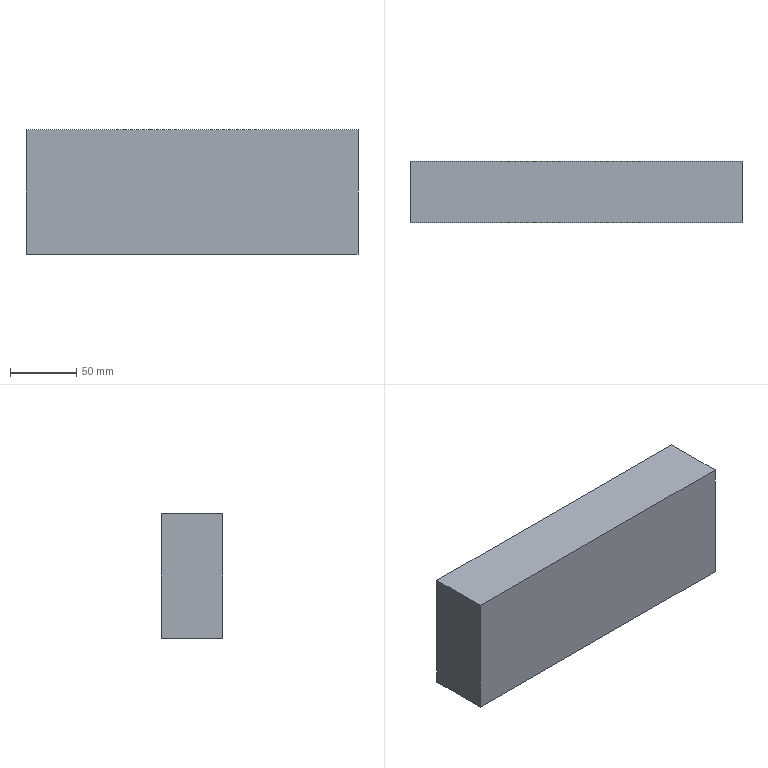Component | SolidWorks | FixedFrame-1 | 1 solid | 22 faces | box 250 x 46.3 x 93.8 mm | volume 1084835 mm3 | plane 14 | cylinder 8 | commonest cylinder face diameters 5 x8
build123d program:
from build123d import *

# Parameters (mm, degrees)
SKETCH2_2_W         = 250
SKETCH2_2_H         = 93.801
BOSS_EXTRUDE1_DEPTH = 44
MOVE_FACE1_BY       = 2.3
SKETCH1_R           = 2.5
CUT_EXTRUDE1_DEPTH  = 8
SKETCH2_W           = 22
SKETCH2_H           = 11
CUT_EXTRUDE2_DEPTH  = 1.5


with BuildPart() as part:
    # Sketch2_2 → Boss-Extrude1 (new body)
    with BuildSketch(Plane.XY):
        with Locations((0, 780.702)):
            Rectangle(SKETCH2_2_W, SKETCH2_2_H)
    extrude(amount=BOSS_EXTRUDE1_DEPTH)

    # Move Face1: a face moved outward by 2.3
    extrude(part.faces().sort_by_distance((0, 780.702, 44))[0], amount=MOVE_FACE1_BY, dir=(0, 0, 1))

    # Sketch1 → Cut-Extrude1 (cut)
    with BuildSketch(Plane.XY.offset(46.3)):
        with Locations((31.25, 802.301)):
            Circle(SKETCH1_R)
        with Locations((31.25, 752.301)):
            Circle(SKETCH1_R)
        with Locations((-31.25, 752.301)):
            Circle(SKETCH1_R)
        with Locations((-31.25, 802.301)):
            Circle(SKETCH1_R)
    extrude(amount=-CUT_EXTRUDE1_DEPTH, mode=Mode.SUBTRACT)

    # Sketch2 → Cut-Extrude2 (cut)
    with BuildSketch(Plane.XY.offset(46.3)):
        with Locations((0, 824.5)):
            Rectangle(SKETCH2_W, SKETCH2_H)
    extrude(amount=-CUT_EXTRUDE2_DEPTH, mode=Mode.SUBTRACT)


solid = part.part

# Placed as in the assembly
solid = solid.moved(Location((0, -295.035, 48), (-90, 0, 0)))
STEP:
#1=CARTESIAN_POINT('',(-1.329,-10.108,-29.697));
#2=VERTEX_POINT('',#1);
#3=CARTESIAN_POINT('',(-1.132,-10.108,-29.697));
#4=VERTEX_POINT('',#3);
#5=CARTESIAN_POINT('',(-1.23,-10.108,-29.697));
#6=DIRECTION('',(0.,1.,0.));
#7=DIRECTION('',(1.,0.,0.));
#8=AXIS2_PLACEMENT_3D('',#5,#6,#7);
#9=CIRCLE('',#8,0.09843);
#10=EDGE_CURVE('',#2,#4,#9,.T.);
#11=ORIENTED_EDGE('',*,*,#10,.F.);
#12=CARTESIAN_POINT('',(-1.329,-9.793,-29.697));
#13=VERTEX_POINT('',#12);
#14=CARTESIAN_POINT('',(-1.329,-10.108,-29.697));
#15=DIRECTION('',(0.,1.,0.));
#16=VECTOR('',#15,39.37);
#17=LINE('',#14,#16);
#18=EDGE_CURVE('',#2,#13,#17,.T.);
#19=ORIENTED_EDGE('',*,*,#18,.T.);
#20=CARTESIAN_POINT('',(-1.132,-9.793,-29.697));
#21=VERTEX_POINT('',#20);
#22=CARTESIAN_POINT('',(-1.23,-9.793,-29.697));
#23=DIRECTION('',(0.,1.,0.));
#24=DIRECTION('',(1.,0.,0.));
#25=AXIS2_PLACEMENT_3D('',#22,#23,#24);
#26=CIRCLE('',#25,0.09843);
#27=EDGE_CURVE('',#13,#21,#26,.T.);
#28=ORIENTED_EDGE('',*,*,#27,.T.);
#29=CARTESIAN_POINT('',(-1.132,-10.108,-29.697));
#30=DIRECTION('',(0.,1.,0.));
#31=VECTOR('',#30,39.37);
#32=LINE('',#29,#31);
#33=EDGE_CURVE('',#4,#21,#32,.T.);
#34=ORIENTED_EDGE('',*,*,#33,.F.);
#35=EDGE_LOOP('',(#11,#19,#28,#34));
#36=FACE_OUTER_BOUND('',#35,.T.);
#37=CARTESIAN_POINT('',(-1.23,-10.108,-29.697));
#38=DIRECTION('',(0.,1.,0.));
#39=DIRECTION('',(1.,0.,0.));
#40=AXIS2_PLACEMENT_3D('',#37,#38,#39);
#41=CYLINDRICAL_SURFACE('',#40,0.09843);
#42=ADVANCED_FACE('',(#36),#41,.F.);
#43=CARTESIAN_POINT('',(-1.329,-10.108,-27.728));
#44=VERTEX_POINT('',#43);
#45=CARTESIAN_POINT('',(-1.132,-10.108,-27.728));
#46=VERTEX_POINT('',#45);
#47=CARTESIAN_POINT('',(-1.23,-10.108,-27.728));
#48=DIRECTION('',(0.,1.,0.));
#49=DIRECTION('',(1.,0.,0.));
#50=AXIS2_PLACEMENT_3D('',#47,#48,#49);
#51=CIRCLE('',#50,0.09843);
#52=EDGE_CURVE('',#44,#46,#51,.T.);
#53=ORIENTED_EDGE('',*,*,#52,.F.);
#54=CARTESIAN_POINT('',(-1.329,-9.793,-27.728));
#55=VERTEX_POINT('',#54);
#56=CARTESIAN_POINT('',(-1.329,-10.108,-27.728));
#57=DIRECTION('',(0.,1.,0.));
#58=VECTOR('',#57,39.37);
#59=LINE('',#56,#58);
#60=EDGE_CURVE('',#44,#55,#59,.T.);
#61=ORIENTED_EDGE('',*,*,#60,.T.);
#62=CARTESIAN_POINT('',(-1.132,-9.793,-27.728));
#63=VERTEX_POINT('',#62);
#64=CARTESIAN_POINT('',(-1.23,-9.793,-27.728));
#65=DIRECTION('',(0.,1.,0.));
#66=DIRECTION('',(1.,0.,0.));
#67=AXIS2_PLACEMENT_3D('',#64,#65,#66);
#68=CIRCLE('',#67,0.09843);
#69=EDGE_CURVE('',#55,#63,#68,.T.);
#70=ORIENTED_EDGE('',*,*,#69,.T.);
#71=CARTESIAN_POINT('',(-1.132,-10.108,-27.728));
#72=DIRECTION('',(0.,1.,0.));
#73=VECTOR('',#72,39.37);
#74=LINE('',#71,#73);
#75=EDGE_CURVE('',#46,#63,#74,.T.);
#76=ORIENTED_EDGE('',*,*,#75,.F.);
#77=EDGE_LOOP('',(#53,#61,#70,#76));
#78=FACE_OUTER_BOUND('',#77,.T.);
#79=CARTESIAN_POINT('',(-1.23,-10.108,-27.728));
#80=DIRECTION('',(0.,1.,0.));
#81=DIRECTION('',(1.,0.,0.));
#82=AXIS2_PLACEMENT_3D('',#79,#80,#81);
#83=CYLINDRICAL_SURFACE('',#82,0.09843);
#84=ADVANCED_FACE('',(#78),#83,.F.);
#85=CARTESIAN_POINT('',(1.132,-10.108,-27.728));
#86=VERTEX_POINT('',#85);
#87=CARTESIAN_POINT('',(1.329,-10.108,-27.728));
#88=VERTEX_POINT('',#87);
#89=CARTESIAN_POINT('',(1.23,-10.108,-27.728));
#90=DIRECTION('',(0.,1.,0.));
#91=DIRECTION('',(1.,0.,0.));
#92=AXIS2_PLACEMENT_3D('',#89,#90,#91);
#93=CIRCLE('',#92,0.09843);
#94=EDGE_CURVE('',#86,#88,#93,.T.);
#95=ORIENTED_EDGE('',*,*,#94,.F.);
#96=CARTESIAN_POINT('',(1.132,-9.793,-27.728));
#97=VERTEX_POINT('',#96);
#98=CARTESIAN_POINT('',(1.132,-10.108,-27.728));
#99=DIRECTION('',(0.,1.,0.));
#100=VECTOR('',#99,39.37);
#101=LINE('',#98,#100);
#102=EDGE_CURVE('',#86,#97,#101,.T.);
#103=ORIENTED_EDGE('',*,*,#102,.T.);
#104=CARTESIAN_POINT('',(1.329,-9.793,-27.728));
#105=VERTEX_POINT('',#104);
#106=CARTESIAN_POINT('',(1.23,-9.793,-27.728));
#107=DIRECTION('',(0.,1.,0.));
#108=DIRECTION('',(1.,0.,0.));
#109=AXIS2_PLACEMENT_3D('',#106,#107,#108);
#110=CIRCLE('',#109,0.09843);
#111=EDGE_CURVE('',#97,#105,#110,.T.);
#112=ORIENTED_EDGE('',*,*,#111,.T.);
#113=CARTESIAN_POINT('',(1.329,-10.108,-27.728));
#114=DIRECTION('',(0.,1.,0.));
#115=VECTOR('',#114,39.37);
#116=LINE('',#113,#115);
#117=EDGE_CURVE('',#88,#105,#116,.T.);
#118=ORIENTED_EDGE('',*,*,#117,.F.);
#119=EDGE_LOOP('',(#95,#103,#112,#118));
#120=FACE_OUTER_BOUND('',#119,.T.);
#121=CARTESIAN_POINT('',(1.23,-10.108,-27.728));
#122=DIRECTION('',(0.,1.,0.));
#123=DIRECTION('',(1.,0.,0.));
#124=AXIS2_PLACEMENT_3D('',#121,#122,#123);
#125=CYLINDRICAL_SURFACE('',#124,0.09843);
#126=ADVANCED_FACE('',(#120),#125,.F.);
#127=CARTESIAN_POINT('',(1.132,-10.108,-29.697));
#128=VERTEX_POINT('',#127);
#129=CARTESIAN_POINT('',(1.329,-10.108,-29.697));
#130=VERTEX_POINT('',#129);
#131=CARTESIAN_POINT('',(1.23,-10.108,-29.697));
#132=DIRECTION('',(0.,1.,0.));
#133=DIRECTION('',(1.,0.,0.));
#134=AXIS2_PLACEMENT_3D('',#131,#132,#133);
#135=CIRCLE('',#134,0.09843);
#136=EDGE_CURVE('',#128,#130,#135,.T.);
#137=ORIENTED_EDGE('',*,*,#136,.F.);
#138=CARTESIAN_POINT('',(1.132,-9.793,-29.697));
#139=VERTEX_POINT('',#138);
#140=CARTESIAN_POINT('',(1.132,-10.108,-29.697));
#141=DIRECTION('',(0.,1.,0.));
#142=VECTOR('',#141,39.37);
#143=LINE('',#140,#142);
#144=EDGE_CURVE('',#128,#139,#143,.T.);
#145=ORIENTED_EDGE('',*,*,#144,.T.);
#146=CARTESIAN_POINT('',(1.329,-9.793,-29.697));
#147=VERTEX_POINT('',#146);
#148=CARTESIAN_POINT('',(1.23,-9.793,-29.697));
#149=DIRECTION('',(0.,1.,0.));
#150=DIRECTION('',(1.,0.,0.));
#151=AXIS2_PLACEMENT_3D('',#148,#149,#150);
#152=CIRCLE('',#151,0.09843);
#153=EDGE_CURVE('',#139,#147,#152,.T.);
#154=ORIENTED_EDGE('',*,*,#153,.T.);
#155=CARTESIAN_POINT('',(1.329,-10.108,-29.697));
#156=DIRECTION('',(0.,1.,0.));
#157=VECTOR('',#156,39.37);
#158=LINE('',#155,#157);
#159=EDGE_CURVE('',#130,#147,#158,.T.);
#160=ORIENTED_EDGE('',*,*,#159,.F.);
#161=EDGE_LOOP('',(#137,#145,#154,#160));
#162=FACE_OUTER_BOUND('',#161,.T.);
#163=CARTESIAN_POINT('',(1.23,-10.108,-29.697));
#164=DIRECTION('',(0.,1.,0.));
#165=DIRECTION('',(1.,0.,0.));
#166=AXIS2_PLACEMENT_3D('',#163,#164,#165);
#167=CYLINDRICAL_SURFACE('',#166,0.09843);
#168=ADVANCED_FACE('',(#162),#167,.F.);
#169=CARTESIAN_POINT('',(4.921,-11.616,-27.));
#170=VERTEX_POINT('',#169);
#171=CARTESIAN_POINT('',(4.921,-11.616,-30.693));
#172=VERTEX_POINT('',#171);
#173=CARTESIAN_POINT('',(4.921,-11.616,-27.));
#174=DIRECTION('',(0.,0.,-1.));
#175=VECTOR('',#174,39.37);
#176=LINE('',#173,#175);
#177=EDGE_CURVE('',#170,#172,#176,.T.);
#178=ORIENTED_EDGE('',*,*,#177,.T.);
#179=CARTESIAN_POINT('',(4.921,-9.793,-30.693));
#180=VERTEX_POINT('',#179);
#181=CARTESIAN_POINT('',(4.921,-9.883,-30.693));
#182=DIRECTION('',(0.,-1.,0.));
#183=VECTOR('',#182,39.37);
#184=LINE('',#181,#183);
#185=EDGE_CURVE('',#180,#172,#184,.T.);
#186=ORIENTED_EDGE('',*,*,#185,.F.);
#187=CARTESIAN_POINT('',(4.921,-9.793,-27.));
#188=VERTEX_POINT('',#187);
#189=CARTESIAN_POINT('',(4.921,-9.793,-27.));
#190=DIRECTION('',(0.,0.,-1.));
#191=VECTOR('',#190,39.37);
#192=LINE('',#189,#191);
#193=EDGE_CURVE('',#188,#180,#192,.T.);
#194=ORIENTED_EDGE('',*,*,#193,.F.);
#195=CARTESIAN_POINT('',(4.921,-9.883,-27.));
#196=DIRECTION('',(0.,-1.,0.));
#197=VECTOR('',#196,39.37);
#198=LINE('',#195,#197);
#199=EDGE_CURVE('',#188,#170,#198,.T.);
#200=ORIENTED_EDGE('',*,*,#199,.T.);
#201=EDGE_LOOP('',(#178,#186,#194,#200));
#202=FACE_OUTER_BOUND('',#201,.T.);
#203=CARTESIAN_POINT('',(4.921,-9.883,-27.));
#204=DIRECTION('',(-1.,0.,0.));
#205=DIRECTION('',(0.,1.,0.));
#206=AXIS2_PLACEMENT_3D('',#203,#204,#205);
#207=PLANE('',#206);
#208=ADVANCED_FACE('',(#202),#207,.F.);
#209=CARTESIAN_POINT('',(-0.4331,-9.793,-30.693));
#210=VERTEX_POINT('',#209);
#211=CARTESIAN_POINT('',(-4.921,-9.793,-30.693));
#212=VERTEX_POINT('',#211);
#213=CARTESIAN_POINT('',(4.921,-9.793,-30.693));
#214=DIRECTION('',(-1.,0.,0.));
#215=VECTOR('',#214,39.37);
#216=LINE('',#213,#215);
#217=EDGE_CURVE('',#210,#212,#216,.T.);
#218=ORIENTED_EDGE('',*,*,#217,.F.);
#219=CARTESIAN_POINT('',(-0.4331,-9.852,-30.693));
#220=VERTEX_POINT('',#219);
#221=CARTESIAN_POINT('',(-0.4331,-9.883,-30.693));
#222=DIRECTION('',(0.,-1.,0.));
#223=VECTOR('',#222,39.37);
#224=LINE('',#221,#223);
#225=EDGE_CURVE('',#210,#220,#224,.T.);
#226=ORIENTED_EDGE('',*,*,#225,.T.);
#227=CARTESIAN_POINT('',(0.4331,-9.852,-30.693));
#228=VERTEX_POINT('',#227);
#229=CARTESIAN_POINT('',(4.921,-9.852,-30.693));
#230=DIRECTION('',(1.,0.,0.));
#231=VECTOR('',#230,39.37);
#232=LINE('',#229,#231);
#233=EDGE_CURVE('',#220,#228,#232,.T.);
#234=ORIENTED_EDGE('',*,*,#233,.T.);
#235=CARTESIAN_POINT('',(0.4331,-9.793,-30.693));
#236=VERTEX_POINT('',#235);
#237=CARTESIAN_POINT('',(0.4331,-9.883,-30.693));
#238=DIRECTION('',(0.,1.,0.));
#239=VECTOR('',#238,39.37);
#240=LINE('',#237,#239);
#241=EDGE_CURVE('',#228,#236,#240,.T.);
#242=ORIENTED_EDGE('',*,*,#241,.T.);
#243=CARTESIAN_POINT('',(4.921,-9.793,-30.693));
#244=DIRECTION('',(-1.,0.,0.));
#245=VECTOR('',#244,39.37);
#246=LINE('',#243,#245);
#247=EDGE_CURVE('',#180,#236,#246,.T.);
#248=ORIENTED_EDGE('',*,*,#247,.F.);
#249=ORIENTED_EDGE('',*,*,#185,.T.);
#250=CARTESIAN_POINT('',(-4.921,-11.616,-30.693));
#251=VERTEX_POINT('',#250);
#252=CARTESIAN_POINT('',(4.921,-11.616,-30.693));
#253=DIRECTION('',(-1.,0.,0.));
#254=VECTOR('',#253,39.37);
#255=LINE('',#252,#254);
#256=EDGE_CURVE('',#172,#251,#255,.T.);
#257=ORIENTED_EDGE('',*,*,#256,.T.);
#258=CARTESIAN_POINT('',(-4.921,-9.883,-30.693));
#259=DIRECTION('',(0.,-1.,0.));
#260=VECTOR('',#259,39.37);
#261=LINE('',#258,#260);
#262=EDGE_CURVE('',#212,#251,#261,.T.);
#263=ORIENTED_EDGE('',*,*,#262,.F.);
#264=EDGE_LOOP('',(#218,#226,#234,#242,#248,#249,#257,#263));
#265=FACE_OUTER_BOUND('',#264,.T.);
#266=CARTESIAN_POINT('',(4.921,-9.883,-30.693));
#267=DIRECTION('',(0.,0.,1.));
#268=DIRECTION('',(0.,-1.,0.));
#269=AXIS2_PLACEMENT_3D('',#266,#267,#268);
#270=PLANE('',#269);
#271=ADVANCED_FACE('',(#265),#270,.F.);
#272=CARTESIAN_POINT('',(-4.921,-11.616,-27.));
#273=VERTEX_POINT('',#272);
#274=CARTESIAN_POINT('',(-4.921,-11.616,-27.));
#275=DIRECTION('',(0.,0.,1.));
#276=VECTOR('',#275,39.37);
#277=LINE('',#274,#276);
#278=EDGE_CURVE('',#251,#273,#277,.T.);
#279=ORIENTED_EDGE('',*,*,#278,.T.);
#280=CARTESIAN_POINT('',(-4.921,-9.793,-27.));
#281=VERTEX_POINT('',#280);
#282=CARTESIAN_POINT('',(-4.921,-9.883,-27.));
#283=DIRECTION('',(0.,-1.,0.));
#284=VECTOR('',#283,39.37);
#285=LINE('',#282,#284);
#286=EDGE_CURVE('',#281,#273,#285,.T.);
#287=ORIENTED_EDGE('',*,*,#286,.F.);
#288=CARTESIAN_POINT('',(-4.921,-9.793,-27.));
#289=DIRECTION('',(0.,0.,1.));
#290=VECTOR('',#289,39.37);
#291=LINE('',#288,#290);
#292=EDGE_CURVE('',#212,#281,#291,.T.);
#293=ORIENTED_EDGE('',*,*,#292,.F.);
#294=ORIENTED_EDGE('',*,*,#262,.T.);
#295=EDGE_LOOP('',(#279,#287,#293,#294));
#296=FACE_OUTER_BOUND('',#295,.T.);
#297=CARTESIAN_POINT('',(-4.921,-9.883,-27.));
#298=DIRECTION('',(1.,0.,0.));
#299=DIRECTION('',(0.,-1.,0.));
#300=AXIS2_PLACEMENT_3D('',#297,#298,#299);
#301=PLANE('',#300);
#302=ADVANCED_FACE('',(#296),#301,.F.);
#303=CARTESIAN_POINT('',(4.921,-11.616,-27.));
#304=DIRECTION('',(1.,0.,0.));
#305=VECTOR('',#304,39.37);
#306=LINE('',#303,#305);
#307=EDGE_CURVE('',#273,#170,#306,.T.);
#308=ORIENTED_EDGE('',*,*,#307,.T.);
#309=ORIENTED_EDGE('',*,*,#199,.F.);
#310=CARTESIAN_POINT('',(4.921,-9.793,-27.));
#311=DIRECTION('',(1.,0.,0.));
#312=VECTOR('',#311,39.37);
#313=LINE('',#310,#312);
#314=EDGE_CURVE('',#281,#188,#313,.T.);
#315=ORIENTED_EDGE('',*,*,#314,.F.);
#316=ORIENTED_EDGE('',*,*,#286,.T.);
#317=EDGE_LOOP('',(#308,#309,#315,#316));
#318=FACE_OUTER_BOUND('',#317,.T.);
#319=CARTESIAN_POINT('',(4.921,-9.883,-27.));
#320=DIRECTION('',(0.,0.,-1.));
#321=DIRECTION('',(0.,1.,0.));
#322=AXIS2_PLACEMENT_3D('',#319,#320,#321);
#323=PLANE('',#322);
#324=ADVANCED_FACE('',(#318),#323,.F.);
#325=CARTESIAN_POINT('',(-0.4331,-9.793,-30.354));
#326=VERTEX_POINT('',#325);
#327=CARTESIAN_POINT('',(-0.4331,-9.793,-30.354));
#328=DIRECTION('',(0.,0.,1.));
#329=VECTOR('',#328,39.37);
#330=LINE('',#327,#329);
#331=EDGE_CURVE('',#210,#326,#330,.T.);
#332=ORIENTED_EDGE('',*,*,#331,.F.);
#333=ORIENTED_EDGE('',*,*,#217,.T.);
#334=ORIENTED_EDGE('',*,*,#292,.T.);
#335=ORIENTED_EDGE('',*,*,#314,.T.);
#336=ORIENTED_EDGE('',*,*,#193,.T.);
#337=ORIENTED_EDGE('',*,*,#247,.T.);
#338=CARTESIAN_POINT('',(0.4331,-9.793,-30.354));
#339=VERTEX_POINT('',#338);
#340=CARTESIAN_POINT('',(0.4331,-9.793,-30.354));
#341=DIRECTION('',(0.,0.,-1.));
#342=VECTOR('',#341,39.37);
#343=LINE('',#340,#342);
#344=EDGE_CURVE('',#339,#236,#343,.T.);
#345=ORIENTED_EDGE('',*,*,#344,.F.);
#346=CARTESIAN_POINT('',(-0.4331,-9.793,-30.354));
#347=DIRECTION('',(1.,0.,0.));
#348=VECTOR('',#347,39.37);
#349=LINE('',#346,#348);
#350=EDGE_CURVE('',#326,#339,#349,.T.);
#351=ORIENTED_EDGE('',*,*,#350,.F.);
#352=EDGE_LOOP('',(#332,#333,#334,#335,#336,#337,#345,#351));
#353=FACE_OUTER_BOUND('',#352,.T.);
#354=CARTESIAN_POINT('',(-1.23,-9.793,-29.697));
#355=DIRECTION('',(0.,1.,0.));
#356=DIRECTION('',(1.,0.,0.));
#357=AXIS2_PLACEMENT_3D('',#354,#355,#356);
#358=CIRCLE('',#357,0.09843);
#359=EDGE_CURVE('',#21,#13,#358,.T.);
#360=ORIENTED_EDGE('',*,*,#359,.F.);
#361=ORIENTED_EDGE('',*,*,#27,.F.);
#362=EDGE_LOOP('',(#360,#361));
#363=FACE_BOUND('',#362,.T.);
#364=CARTESIAN_POINT('',(-1.23,-9.793,-27.728));
#365=DIRECTION('',(0.,1.,0.));
#366=DIRECTION('',(1.,0.,0.));
#367=AXIS2_PLACEMENT_3D('',#364,#365,#366);
#368=CIRCLE('',#367,0.09843);
#369=EDGE_CURVE('',#63,#55,#368,.T.);
#370=ORIENTED_EDGE('',*,*,#369,.F.);
#371=ORIENTED_EDGE('',*,*,#69,.F.);
#372=EDGE_LOOP('',(#370,#371));
#373=FACE_BOUND('',#372,.T.);
#374=CARTESIAN_POINT('',(1.23,-9.793,-27.728));
#375=DIRECTION('',(0.,1.,0.));
#376=DIRECTION('',(1.,0.,0.));
#377=AXIS2_PLACEMENT_3D('',#374,#375,#376);
#378=CIRCLE('',#377,0.09843);
#379=EDGE_CURVE('',#105,#97,#378,.T.);
#380=ORIENTED_EDGE('',*,*,#379,.F.);
#381=ORIENTED_EDGE('',*,*,#111,.F.);
#382=EDGE_LOOP('',(#380,#381));
#383=FACE_BOUND('',#382,.T.);
#384=CARTESIAN_POINT('',(1.23,-9.793,-29.697));
#385=DIRECTION('',(0.,1.,0.));
#386=DIRECTION('',(1.,0.,0.));
#387=AXIS2_PLACEMENT_3D('',#384,#385,#386);
#388=CIRCLE('',#387,0.09843);
#389=EDGE_CURVE('',#147,#139,#388,.T.);
#390=ORIENTED_EDGE('',*,*,#389,.F.);
#391=ORIENTED_EDGE('',*,*,#153,.F.);
#392=EDGE_LOOP('',(#390,#391));
#393=FACE_BOUND('',#392,.T.);
#394=CARTESIAN_POINT('',(0.,-9.793,1.89));
#395=DIRECTION('',(0.,1.,0.));
#396=DIRECTION('',(1.,0.,0.));
#397=AXIS2_PLACEMENT_3D('',#394,#395,#396);
#398=PLANE('',#397);
#399=ADVANCED_FACE('',(#353,#363,#373,#383,#393),#398,.T.);
#400=ORIENTED_EDGE('',*,*,#177,.F.);
#401=ORIENTED_EDGE('',*,*,#307,.F.);
#402=ORIENTED_EDGE('',*,*,#278,.F.);
#403=ORIENTED_EDGE('',*,*,#256,.F.);
#404=EDGE_LOOP('',(#400,#401,#402,#403));
#405=FACE_OUTER_BOUND('',#404,.T.);
#406=CARTESIAN_POINT('',(0.,-11.616,1.89));
#407=DIRECTION('',(0.,1.,0.));
#408=DIRECTION('',(1.,0.,0.));
#409=AXIS2_PLACEMENT_3D('',#406,#407,#408);
#410=PLANE('',#409);
#411=ADVANCED_FACE('',(#405),#410,.F.);
#412=ORIENTED_EDGE('',*,*,#144,.F.);
#413=CARTESIAN_POINT('',(1.23,-10.108,-29.697));
#414=DIRECTION('',(0.,1.,0.));
#415=DIRECTION('',(1.,0.,0.));
#416=AXIS2_PLACEMENT_3D('',#413,#414,#415);
#417=CIRCLE('',#416,0.09843);
#418=EDGE_CURVE('',#130,#128,#417,.T.);
#419=ORIENTED_EDGE('',*,*,#418,.F.);
#420=ORIENTED_EDGE('',*,*,#159,.T.);
#421=ORIENTED_EDGE('',*,*,#389,.T.);
#422=EDGE_LOOP('',(#412,#419,#420,#421));
#423=FACE_OUTER_BOUND('',#422,.T.);
#424=CARTESIAN_POINT('',(1.23,-10.108,-29.697));
#425=DIRECTION('',(0.,1.,0.));
#426=DIRECTION('',(1.,0.,0.));
#427=AXIS2_PLACEMENT_3D('',#424,#425,#426);
#428=CYLINDRICAL_SURFACE('',#427,0.09843);
#429=ADVANCED_FACE('',(#423),#428,.F.);
#430=ORIENTED_EDGE('',*,*,#418,.T.);
#431=ORIENTED_EDGE('',*,*,#136,.T.);
#432=EDGE_LOOP('',(#430,#431));
#433=FACE_OUTER_BOUND('',#432,.T.);
#434=CARTESIAN_POINT('',(1.23,-10.108,-29.697));
#435=DIRECTION('',(0.,1.,0.));
#436=DIRECTION('',(1.,0.,0.));
#437=AXIS2_PLACEMENT_3D('',#434,#435,#436);
#438=PLANE('',#437);
#439=ADVANCED_FACE('',(#433),#438,.T.);
#440=ORIENTED_EDGE('',*,*,#102,.F.);
#441=CARTESIAN_POINT('',(1.23,-10.108,-27.728));
#442=DIRECTION('',(0.,1.,0.));
#443=DIRECTION('',(1.,0.,0.));
#444=AXIS2_PLACEMENT_3D('',#441,#442,#443);
#445=CIRCLE('',#444,0.09843);
#446=EDGE_CURVE('',#88,#86,#445,.T.);
#447=ORIENTED_EDGE('',*,*,#446,.F.);
#448=ORIENTED_EDGE('',*,*,#117,.T.);
#449=ORIENTED_EDGE('',*,*,#379,.T.);
#450=EDGE_LOOP('',(#440,#447,#448,#449));
#451=FACE_OUTER_BOUND('',#450,.T.);
#452=CARTESIAN_POINT('',(1.23,-10.108,-27.728));
#453=DIRECTION('',(0.,1.,0.));
#454=DIRECTION('',(1.,0.,0.));
#455=AXIS2_PLACEMENT_3D('',#452,#453,#454);
#456=CYLINDRICAL_SURFACE('',#455,0.09843);
#457=ADVANCED_FACE('',(#451),#456,.F.);
#458=ORIENTED_EDGE('',*,*,#446,.T.);
#459=ORIENTED_EDGE('',*,*,#94,.T.);
#460=EDGE_LOOP('',(#458,#459));
#461=FACE_OUTER_BOUND('',#460,.T.);
#462=CARTESIAN_POINT('',(1.23,-10.108,-27.728));
#463=DIRECTION('',(0.,1.,0.));
#464=DIRECTION('',(1.,0.,0.));
#465=AXIS2_PLACEMENT_3D('',#462,#463,#464);
#466=PLANE('',#465);
#467=ADVANCED_FACE('',(#461),#466,.T.);
#468=ORIENTED_EDGE('',*,*,#60,.F.);
#469=CARTESIAN_POINT('',(-1.23,-10.108,-27.728));
#470=DIRECTION('',(0.,1.,0.));
#471=DIRECTION('',(1.,0.,0.));
#472=AXIS2_PLACEMENT_3D('',#469,#470,#471);
#473=CIRCLE('',#472,0.09843);
#474=EDGE_CURVE('',#46,#44,#473,.T.);
#475=ORIENTED_EDGE('',*,*,#474,.F.);
#476=ORIENTED_EDGE('',*,*,#75,.T.);
#477=ORIENTED_EDGE('',*,*,#369,.T.);
#478=EDGE_LOOP('',(#468,#475,#476,#477));
#479=FACE_OUTER_BOUND('',#478,.T.);
#480=CARTESIAN_POINT('',(-1.23,-10.108,-27.728));
#481=DIRECTION('',(0.,1.,0.));
#482=DIRECTION('',(1.,0.,0.));
#483=AXIS2_PLACEMENT_3D('',#480,#481,#482);
#484=CYLINDRICAL_SURFACE('',#483,0.09843);
#485=ADVANCED_FACE('',(#479),#484,.F.);
#486=ORIENTED_EDGE('',*,*,#474,.T.);
#487=ORIENTED_EDGE('',*,*,#52,.T.);
#488=EDGE_LOOP('',(#486,#487));
#489=FACE_OUTER_BOUND('',#488,.T.);
#490=CARTESIAN_POINT('',(-1.23,-10.108,-27.728));
#491=DIRECTION('',(0.,1.,0.));
#492=DIRECTION('',(1.,0.,0.));
#493=AXIS2_PLACEMENT_3D('',#490,#491,#492);
#494=PLANE('',#493);
#495=ADVANCED_FACE('',(#489),#494,.T.);
#496=ORIENTED_EDGE('',*,*,#18,.F.);
#497=CARTESIAN_POINT('',(-1.23,-10.108,-29.697));
#498=DIRECTION('',(0.,1.,0.));
#499=DIRECTION('',(1.,0.,0.));
#500=AXIS2_PLACEMENT_3D('',#497,#498,#499);
#501=CIRCLE('',#500,0.09843);
#502=EDGE_CURVE('',#4,#2,#501,.T.);
#503=ORIENTED_EDGE('',*,*,#502,.F.);
#504=ORIENTED_EDGE('',*,*,#33,.T.);
#505=ORIENTED_EDGE('',*,*,#359,.T.);
#506=EDGE_LOOP('',(#496,#503,#504,#505));
#507=FACE_OUTER_BOUND('',#506,.T.);
#508=CARTESIAN_POINT('',(-1.23,-10.108,-29.697));
#509=DIRECTION('',(0.,1.,0.));
#510=DIRECTION('',(1.,0.,0.));
#511=AXIS2_PLACEMENT_3D('',#508,#509,#510);
#512=CYLINDRICAL_SURFACE('',#511,0.09843);
#513=ADVANCED_FACE('',(#507),#512,.F.);
#514=ORIENTED_EDGE('',*,*,#502,.T.);
#515=ORIENTED_EDGE('',*,*,#10,.T.);
#516=EDGE_LOOP('',(#514,#515));
#517=FACE_OUTER_BOUND('',#516,.T.);
#518=CARTESIAN_POINT('',(-1.23,-10.108,-29.697));
#519=DIRECTION('',(0.,1.,0.));
#520=DIRECTION('',(1.,0.,0.));
#521=AXIS2_PLACEMENT_3D('',#518,#519,#520);
#522=PLANE('',#521);
#523=ADVANCED_FACE('',(#517),#522,.T.);
#524=ORIENTED_EDGE('',*,*,#331,.T.);
#525=CARTESIAN_POINT('',(-0.4331,-9.852,-30.354));
#526=VERTEX_POINT('',#525);
#527=CARTESIAN_POINT('',(-0.4331,-9.852,-30.354));
#528=DIRECTION('',(0.,1.,0.));
#529=VECTOR('',#528,39.37);
#530=LINE('',#527,#529);
#531=EDGE_CURVE('',#526,#326,#530,.T.);
#532=ORIENTED_EDGE('',*,*,#531,.F.);
#533=CARTESIAN_POINT('',(-0.4331,-9.852,-30.354));
#534=DIRECTION('',(0.,0.,1.));
#535=VECTOR('',#534,39.37);
#536=LINE('',#533,#535);
#537=EDGE_CURVE('',#220,#526,#536,.T.);
#538=ORIENTED_EDGE('',*,*,#537,.F.);
#539=ORIENTED_EDGE('',*,*,#225,.F.);
#540=EDGE_LOOP('',(#524,#532,#538,#539));
#541=FACE_OUTER_BOUND('',#540,.T.);
#542=CARTESIAN_POINT('',(-0.4331,-9.852,-30.354));
#543=DIRECTION('',(-1.,0.,0.));
#544=DIRECTION('',(0.,1.,0.));
#545=AXIS2_PLACEMENT_3D('',#542,#543,#544);
#546=PLANE('',#545);
#547=ADVANCED_FACE('',(#541),#546,.F.);
#548=CARTESIAN_POINT('',(0.4331,-9.852,-30.354));
#549=VERTEX_POINT('',#548);
#550=CARTESIAN_POINT('',(0.4331,-9.852,-30.354));
#551=DIRECTION('',(0.,0.,-1.));
#552=VECTOR('',#551,39.37);
#553=LINE('',#550,#552);
#554=EDGE_CURVE('',#549,#228,#553,.T.);
#555=ORIENTED_EDGE('',*,*,#554,.F.);
#556=CARTESIAN_POINT('',(0.4331,-9.852,-30.354));
#557=DIRECTION('',(0.,1.,0.));
#558=VECTOR('',#557,39.37);
#559=LINE('',#556,#558);
#560=EDGE_CURVE('',#549,#339,#559,.T.);
#561=ORIENTED_EDGE('',*,*,#560,.T.);
#562=ORIENTED_EDGE('',*,*,#344,.T.);
#563=ORIENTED_EDGE('',*,*,#241,.F.);
#564=EDGE_LOOP('',(#555,#561,#562,#563));
#565=FACE_OUTER_BOUND('',#564,.T.);
#566=CARTESIAN_POINT('',(0.4331,-9.852,-30.354));
#567=DIRECTION('',(1.,0.,0.));
#568=DIRECTION('',(0.,-1.,0.));
#569=AXIS2_PLACEMENT_3D('',#566,#567,#568);
#570=PLANE('',#569);
#571=ADVANCED_FACE('',(#565),#570,.F.);
#572=ORIENTED_EDGE('',*,*,#537,.T.);
#573=CARTESIAN_POINT('',(-0.4331,-9.852,-30.354));
#574=DIRECTION('',(1.,0.,0.));
#575=VECTOR('',#574,39.37);
#576=LINE('',#573,#575);
#577=EDGE_CURVE('',#526,#549,#576,.T.);
#578=ORIENTED_EDGE('',*,*,#577,.T.);
#579=ORIENTED_EDGE('',*,*,#554,.T.);
#580=ORIENTED_EDGE('',*,*,#233,.F.);
#581=EDGE_LOOP('',(#572,#578,#579,#580));
#582=FACE_OUTER_BOUND('',#581,.T.);
#583=CARTESIAN_POINT('',(0.,-9.852,1.89));
#584=DIRECTION('',(0.,-1.,0.));
#585=DIRECTION('',(-1.,0.,0.));
#586=AXIS2_PLACEMENT_3D('',#583,#584,#585);
#587=PLANE('',#586);
#588=ADVANCED_FACE('',(#582),#587,.F.);
#589=ORIENTED_EDGE('',*,*,#350,.T.);
#590=ORIENTED_EDGE('',*,*,#560,.F.);
#591=ORIENTED_EDGE('',*,*,#577,.F.);
#592=ORIENTED_EDGE('',*,*,#531,.T.);
#593=EDGE_LOOP('',(#589,#590,#591,#592));
#594=FACE_OUTER_BOUND('',#593,.T.);
#595=CARTESIAN_POINT('',(-0.4331,-9.852,-30.354));
#596=DIRECTION('',(0.,0.,1.));
#597=DIRECTION('',(0.,-1.,0.));
#598=AXIS2_PLACEMENT_3D('',#595,#596,#597);
#599=PLANE('',#598);
#600=ADVANCED_FACE('',(#594),#599,.F.);
#601=CLOSED_SHELL('',(#42,#84,#126,#168,#208,#271,#302,#324,#399,#411,#429,#439,#457,#467,#485,#495,#513,#523,#547,#571,#588,#600));
#602=MANIFOLD_SOLID_BREP('',#601);
#603=CARTESIAN_POINT('',(0.,0.,0.));
#604=DIRECTION('',(0.,0.,1.));
#605=DIRECTION('',(1.,0.,0.));
#606=AXIS2_PLACEMENT_3D('',#603,#604,#605);
#607=(LENGTH_UNIT()NAMED_UNIT(*)SI_UNIT($,.METRE.));
#608=LENGTH_MEASURE_WITH_UNIT(LENGTH_MEASURE(0.0254),#607);
#609=DIMENSIONAL_EXPONENTS(1.,0.,0.,0.,0.,0.,0.);
#610=(CONVERSION_BASED_UNIT('',#608)LENGTH_UNIT()NAMED_UNIT(#609));
#611=UNCERTAINTY_MEASURE_WITH_UNIT(LENGTH_MEASURE(0.00001),#610,'','');
#612=(NAMED_UNIT(*)PLANE_ANGLE_UNIT()SI_UNIT($,.RADIAN.));
#613=(NAMED_UNIT(*)SI_UNIT($,.STERADIAN.)SOLID_ANGLE_UNIT());
#614=(GEOMETRIC_REPRESENTATION_CONTEXT(3)GLOBAL_UNCERTAINTY_ASSIGNED_CONTEXT((#611))GLOBAL_UNIT_ASSIGNED_CONTEXT((#610,#612,#613))REPRESENTATION_CONTEXT('',''));
#615=ADVANCED_BREP_SHAPE_REPRESENTATION('',(#602,#606),#614);
#616=COLOUR_RGB('',0.7922,0.8196,0.9333);
#617=FILL_AREA_STYLE_COLOUR('',#616);
#618=FILL_AREA_STYLE('',(#617));
#619=SURFACE_STYLE_FILL_AREA(#618);
#620=SURFACE_SIDE_STYLE('',(#619));
#621=SURFACE_STYLE_USAGE(.BOTH.,#620);
#622=PRESENTATION_STYLE_ASSIGNMENT((#621));
#623=STYLED_ITEM('',(#622),#602);
#624=PRESENTATION_LAYER_ASSIGNMENT('','',(#623));
#625=(LENGTH_UNIT()NAMED_UNIT(*)SI_UNIT($,.METRE.));
#626=LENGTH_MEASURE_WITH_UNIT(LENGTH_MEASURE(0.0254),#625);
#627=DIMENSIONAL_EXPONENTS(1.,0.,0.,0.,0.,0.,0.);
#628=(CONVERSION_BASED_UNIT('',#626)LENGTH_UNIT()NAMED_UNIT(#627));
#629=UNCERTAINTY_MEASURE_WITH_UNIT(LENGTH_MEASURE(0.00001),#628,'','');
#630=(NAMED_UNIT(*)PLANE_ANGLE_UNIT()SI_UNIT($,.RADIAN.));
#631=(NAMED_UNIT(*)SI_UNIT($,.STERADIAN.)SOLID_ANGLE_UNIT());
#632=(GEOMETRIC_REPRESENTATION_CONTEXT(3)GLOBAL_UNCERTAINTY_ASSIGNED_CONTEXT((#629))GLOBAL_UNIT_ASSIGNED_CONTEXT((#628,#630,#631))REPRESENTATION_CONTEXT('',''));
#633=MECHANICAL_DESIGN_GEOMETRIC_PRESENTATION_REPRESENTATION('',(#623),#632);